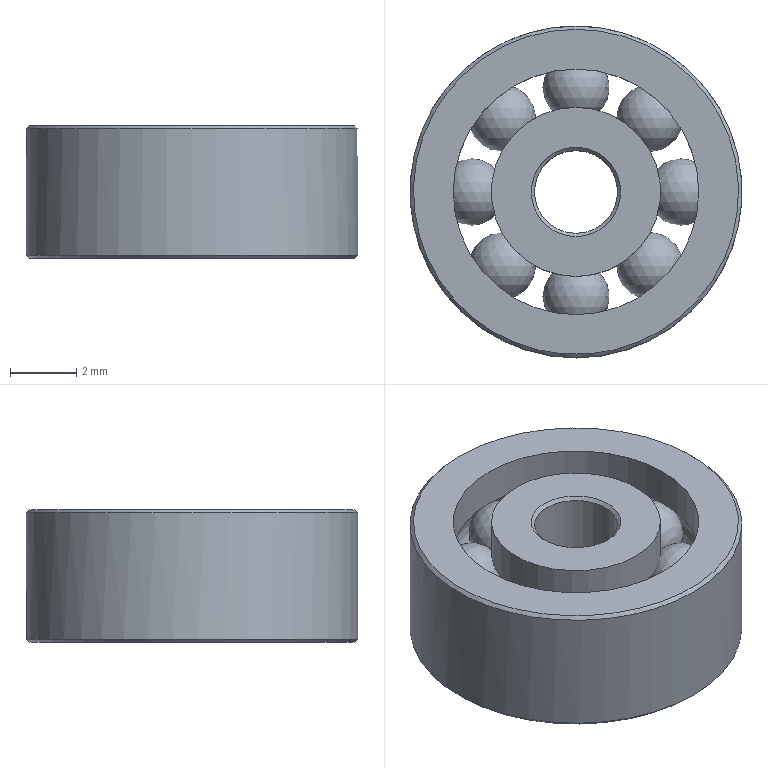Component | NX | BEARING | 10 solids | 24 faces | volume 218 mm3 | sphere 8 | cylinder 6 | plane 4 | cone 4 | torus 2 | commonest cylinder face diameters 7.4 x2 5.1 x2 10 x1 2.5 x1